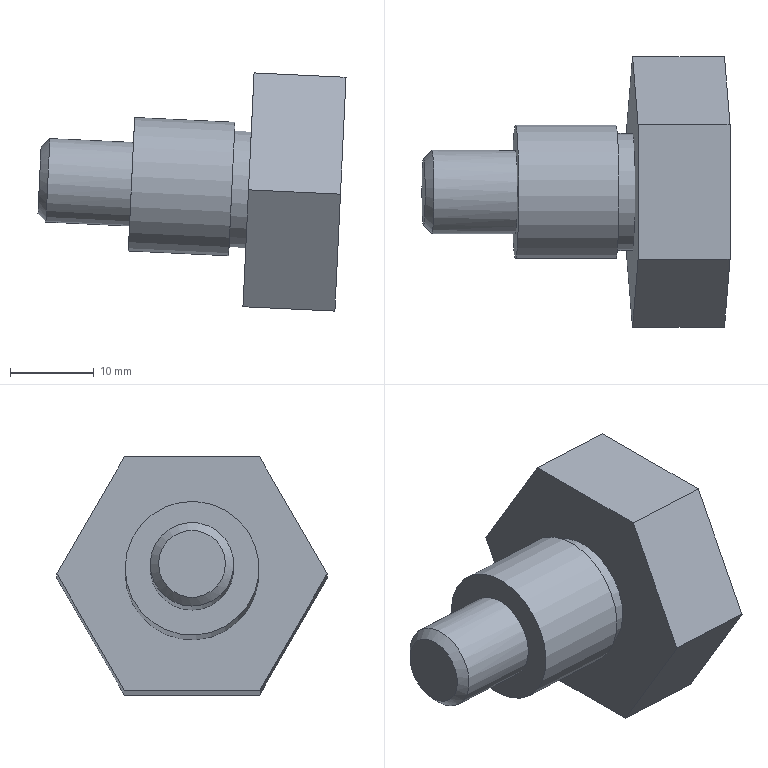Component | NX | SMALL_SHAFT | 1 solid | 15 faces | box 36.81 x 32.3 x 28.46 mm | volume 11024 mm3 | plane 11 | cylinder 3 | cone 1 | commonest cylinder face diameters 16 x1 10 x1 14 x1
STEP:
#1=CARTESIAN_POINT('',(0.,0.,0.));
#2=DIRECTION('',(0.,0.,1.));
#3=DIRECTION('',(1.,0.,0.));
#4=AXIS2_PLACEMENT_3D('',#1,#2,#3);
#5=CARTESIAN_POINT('',(20.177,-44.911,-1.909));
#6=VERTEX_POINT('',#5);
#7=CARTESIAN_POINT('',(20.507,-56.911,5.011));
#8=VERTEX_POINT('',#7);
#9=CARTESIAN_POINT('',(20.177,-52.911,-1.909));
#10=DIRECTION('',(-0.9989,0.,0.04757));
#11=DIRECTION('',(0.,1.,0.));
#12=AXIS2_PLACEMENT_3D('',#9,#10,#11);
#13=CIRCLE('',#12,8.);
#14=CARTESIAN_POINT('',(8.191,-52.911,-1.338));
#15=DIRECTION('',(0.9989,0.,-0.04757));
#16=DIRECTION('',(0.,-1.,0.));
#17=AXIS2_PLACEMENT_3D('',#14,#15,#16);
#18=CYLINDRICAL_SURFACE('',#17,8.);
#19=CARTESIAN_POINT('',(9.425,12.));
#20=DIRECTION('',(-1.,0.));
#21=VECTOR('',#20,1.);
#22=LINE('',#19,#21);
#23=(GEOMETRIC_REPRESENTATION_CONTEXT(2)PARAMETRIC_REPRESENTATION_CONTEXT()REPRESENTATION_CONTEXT('',''));
#24=DEFINITIONAL_REPRESENTATION('',(#22),#23);
#25=PCURVE('',#18,#24);
#26=CARTESIAN_POINT('',(20.51,-52.911,5.083));
#27=DIRECTION('',(-0.9989,0.,0.04757));
#28=DIRECTION('',(0.,1.,0.));
#29=AXIS2_PLACEMENT_3D('',#26,#27,#28);
#30=PLANE('',#29);
#31=CARTESIAN_POINT('',(0.,7.));
#32=DIRECTION('',(1.,0.));
#33=AXIS2_PLACEMENT_2D('',#31,#32);
#34=CIRCLE('',#33,8.);
#35=(GEOMETRIC_REPRESENTATION_CONTEXT(2)PARAMETRIC_REPRESENTATION_CONTEXT()REPRESENTATION_CONTEXT('',''));
#36=DEFINITIONAL_REPRESENTATION('',(#34),#35);
#37=PCURVE('',#30,#36);
#38=SURFACE_CURVE('',#13,(#25,#37),.PCURVE_S1.);
#39=EDGE_CURVE('',#6,#8,#38,.T.);
#40=ORIENTED_EDGE('',*,*,#39,.T.);
#41=CARTESIAN_POINT('',(8.521,-56.911,5.582));
#42=VERTEX_POINT('',#41);
#43=CARTESIAN_POINT('',(8.521,-56.911,5.582));
#44=CARTESIAN_POINT('',(20.507,-56.911,5.011));
#45=B_SPLINE_CURVE_WITH_KNOTS('',1,(#43,#44),.UNSPECIFIED.,.F.,.F.,(2,2),(0.,12.),.PIECEWISE_BEZIER_KNOTS.);
#46=CARTESIAN_POINT('',(5.236,0.));
#47=DIRECTION('',(0.,1.));
#48=VECTOR('',#47,1.);
#49=LINE('',#46,#48);
#50=(GEOMETRIC_REPRESENTATION_CONTEXT(2)PARAMETRIC_REPRESENTATION_CONTEXT()REPRESENTATION_CONTEXT('',''));
#51=DEFINITIONAL_REPRESENTATION('',(#49),#50);
#52=PCURVE('',#18,#51);
#53=CARTESIAN_POINT('',(11.519,0.));
#54=DIRECTION('',(0.,1.));
#55=VECTOR('',#54,1.);
#56=LINE('',#53,#55);
#57=(GEOMETRIC_REPRESENTATION_CONTEXT(2)PARAMETRIC_REPRESENTATION_CONTEXT()REPRESENTATION_CONTEXT('',''));
#58=DEFINITIONAL_REPRESENTATION('',(#56),#57);
#59=PCURVE('',#18,#58);
#60=SEAM_CURVE('',#45,(#52,#59),.PCURVE_S1.);
#61=EDGE_CURVE('',#42,#8,#60,.T.);
#62=ORIENTED_EDGE('',*,*,#61,.F.);
#63=CARTESIAN_POINT('',(8.191,-52.911,-1.338));
#64=DIRECTION('',(-0.9989,0.,0.04757));
#65=DIRECTION('',(0.0412,-0.5,0.865));
#66=AXIS2_PLACEMENT_3D('',#63,#64,#65);
#67=CIRCLE('',#66,8.);
#68=CARTESIAN_POINT('',(11.519,0.));
#69=DIRECTION('',(-1.,0.));
#70=VECTOR('',#69,1.);
#71=LINE('',#68,#70);
#72=(GEOMETRIC_REPRESENTATION_CONTEXT(2)PARAMETRIC_REPRESENTATION_CONTEXT()REPRESENTATION_CONTEXT('',''));
#73=DEFINITIONAL_REPRESENTATION('',(#71),#72);
#74=PCURVE('',#18,#73);
#75=CARTESIAN_POINT('',(8.191,-52.911,-1.338));
#76=DIRECTION('',(-0.9989,0.,0.04757));
#77=DIRECTION('',(0.,1.,0.));
#78=AXIS2_PLACEMENT_3D('',#75,#76,#77);
#79=PLANE('',#78);
#80=CARTESIAN_POINT('',(0.,0.));
#81=DIRECTION('',(-0.5,-0.866));
#82=AXIS2_PLACEMENT_2D('',#80,#81);
#83=CIRCLE('',#82,8.);
#84=(GEOMETRIC_REPRESENTATION_CONTEXT(2)PARAMETRIC_REPRESENTATION_CONTEXT()REPRESENTATION_CONTEXT('',''));
#85=DEFINITIONAL_REPRESENTATION('',(#83),#84);
#86=PCURVE('',#79,#85);
#87=SURFACE_CURVE('',#67,(#74,#86),.PCURVE_S1.);
#88=EDGE_CURVE('',#42,#42,#87,.T.);
#89=ORIENTED_EDGE('',*,*,#88,.F.);
#90=ORIENTED_EDGE('',*,*,#61,.T.);
#91=CARTESIAN_POINT('',(20.177,-52.911,-1.909));
#92=DIRECTION('',(-0.9989,0.,0.04757));
#93=DIRECTION('',(0.,1.,0.));
#94=AXIS2_PLACEMENT_3D('',#91,#92,#93);
#95=CIRCLE('',#94,8.);
#96=CARTESIAN_POINT('',(15.708,12.));
#97=DIRECTION('',(-1.,0.));
#98=VECTOR('',#97,1.);
#99=LINE('',#96,#98);
#100=(GEOMETRIC_REPRESENTATION_CONTEXT(2)PARAMETRIC_REPRESENTATION_CONTEXT()REPRESENTATION_CONTEXT('',''));
#101=DEFINITIONAL_REPRESENTATION('',(#99),#100);
#102=PCURVE('',#18,#101);
#103=CARTESIAN_POINT('',(0.,7.));
#104=DIRECTION('',(1.,0.));
#105=AXIS2_PLACEMENT_2D('',#103,#104);
#106=CIRCLE('',#105,8.);
#107=(GEOMETRIC_REPRESENTATION_CONTEXT(2)PARAMETRIC_REPRESENTATION_CONTEXT()REPRESENTATION_CONTEXT('',''));
#108=DEFINITIONAL_REPRESENTATION('',(#106),#107);
#109=PCURVE('',#30,#108);
#110=SURFACE_CURVE('',#95,(#102,#109),.PCURVE_S1.);
#111=EDGE_CURVE('',#8,#6,#110,.T.);
#112=ORIENTED_EDGE('',*,*,#111,.T.);
#113=EDGE_LOOP('',(#40,#62,#89,#90,#112));
#114=FACE_BOUND('',#113,.T.);
#115=ADVANCED_FACE('',(#114),#18,.T.);
#116=CARTESIAN_POINT('',(7.953,-52.911,-6.333));
#117=VERTEX_POINT('',#116);
#118=CARTESIAN_POINT('',(8.191,-52.911,-1.338));
#119=DIRECTION('',(-0.9989,0.,0.04757));
#120=DIRECTION('',(-0.04757,0.,-0.9989));
#121=AXIS2_PLACEMENT_3D('',#118,#119,#120);
#122=CIRCLE('',#121,5.);
#123=CARTESIAN_POINT('',(0.,0.));
#124=DIRECTION('',(0.,1.));
#125=AXIS2_PLACEMENT_2D('',#123,#124);
#126=CIRCLE('',#125,5.);
#127=(GEOMETRIC_REPRESENTATION_CONTEXT(2)PARAMETRIC_REPRESENTATION_CONTEXT()REPRESENTATION_CONTEXT('',''));
#128=DEFINITIONAL_REPRESENTATION('',(#126),#127);
#129=PCURVE('',#79,#128);
#130=CARTESIAN_POINT('',(-2.796,-52.911,-0.815));
#131=DIRECTION('',(0.9989,0.,-0.04757));
#132=DIRECTION('',(0.,-1.,0.));
#133=AXIS2_PLACEMENT_3D('',#130,#131,#132);
#134=CYLINDRICAL_SURFACE('',#133,5.);
#135=CARTESIAN_POINT('',(7.854,11.));
#136=DIRECTION('',(-1.,0.));
#137=VECTOR('',#136,1.);
#138=LINE('',#135,#137);
#139=(GEOMETRIC_REPRESENTATION_CONTEXT(2)PARAMETRIC_REPRESENTATION_CONTEXT()REPRESENTATION_CONTEXT('',''));
#140=DEFINITIONAL_REPRESENTATION('',(#138),#139);
#141=PCURVE('',#134,#140);
#142=SURFACE_CURVE('',#122,(#129,#141),.PCURVE_S1.);
#143=EDGE_CURVE('',#117,#117,#142,.T.);
#144=ORIENTED_EDGE('',*,*,#143,.F.);
#145=EDGE_LOOP('',(#144));
#146=FACE_BOUND('',#145,.T.);
#147=ORIENTED_EDGE('',*,*,#88,.T.);
#148=EDGE_LOOP('',(#147));
#149=FACE_BOUND('',#148,.T.);
#150=ADVANCED_FACE('',(#146,#149),#79,.T.);
#151=CARTESIAN_POINT('',(-1.798,-47.911,-0.8626));
#152=VERTEX_POINT('',#151);
#153=CARTESIAN_POINT('',(-2.035,-52.911,-5.857));
#154=VERTEX_POINT('',#153);
#155=CARTESIAN_POINT('',(-1.798,-52.911,-0.8626));
#156=DIRECTION('',(0.9989,0.,-0.04757));
#157=DIRECTION('',(0.,1.,0.));
#158=AXIS2_PLACEMENT_3D('',#155,#156,#157);
#159=CIRCLE('',#158,5.);
#160=CARTESIAN_POINT('',(3.142,1.));
#161=DIRECTION('',(1.,0.));
#162=VECTOR('',#161,1.);
#163=LINE('',#160,#162);
#164=(GEOMETRIC_REPRESENTATION_CONTEXT(2)PARAMETRIC_REPRESENTATION_CONTEXT()REPRESENTATION_CONTEXT('',''));
#165=DEFINITIONAL_REPRESENTATION('',(#163),#164);
#166=PCURVE('',#134,#165);
#167=CARTESIAN_POINT('',(-2.796,-52.911,-0.815));
#168=DIRECTION('',(0.9989,0.,-0.04757));
#169=DIRECTION('',(0.,-1.,0.));
#170=AXIS2_PLACEMENT_3D('',#167,#168,#169);
#171=CONICAL_SURFACE('',#170,4.,0.7854);
#172=CARTESIAN_POINT('',(3.142,1.));
#173=DIRECTION('',(1.,0.));
#174=VECTOR('',#173,1.);
#175=LINE('',#172,#174);
#176=(GEOMETRIC_REPRESENTATION_CONTEXT(2)PARAMETRIC_REPRESENTATION_CONTEXT()REPRESENTATION_CONTEXT('',''));
#177=DEFINITIONAL_REPRESENTATION('',(#175),#176);
#178=PCURVE('',#171,#177);
#179=SURFACE_CURVE('',#159,(#166,#178),.PCURVE_S1.);
#180=EDGE_CURVE('',#152,#154,#179,.T.);
#181=ORIENTED_EDGE('',*,*,#180,.T.);
#182=CARTESIAN_POINT('',(-2.035,-52.911,-5.857));
#183=CARTESIAN_POINT('',(7.953,-52.911,-6.333));
#184=B_SPLINE_CURVE_WITH_KNOTS('',1,(#182,#183),.UNSPECIFIED.,.F.,.F.,(2,2),(1.,11.),.PIECEWISE_BEZIER_KNOTS.);
#185=CARTESIAN_POINT('',(7.854,0.));
#186=DIRECTION('',(0.,1.));
#187=VECTOR('',#186,1.);
#188=LINE('',#185,#187);
#189=(GEOMETRIC_REPRESENTATION_CONTEXT(2)PARAMETRIC_REPRESENTATION_CONTEXT()REPRESENTATION_CONTEXT('',''));
#190=DEFINITIONAL_REPRESENTATION('',(#188),#189);
#191=PCURVE('',#134,#190);
#192=CARTESIAN_POINT('',(1.571,0.));
#193=DIRECTION('',(0.,1.));
#194=VECTOR('',#193,1.);
#195=LINE('',#192,#194);
#196=(GEOMETRIC_REPRESENTATION_CONTEXT(2)PARAMETRIC_REPRESENTATION_CONTEXT()REPRESENTATION_CONTEXT('',''));
#197=DEFINITIONAL_REPRESENTATION('',(#195),#196);
#198=PCURVE('',#134,#197);
#199=SEAM_CURVE('',#184,(#191,#198),.PCURVE_S1.);
#200=EDGE_CURVE('',#154,#117,#199,.T.);
#201=ORIENTED_EDGE('',*,*,#200,.T.);
#202=ORIENTED_EDGE('',*,*,#143,.T.);
#203=ORIENTED_EDGE('',*,*,#200,.F.);
#204=CARTESIAN_POINT('',(-1.798,-52.911,-0.8626));
#205=DIRECTION('',(0.9989,0.,-0.04757));
#206=DIRECTION('',(0.,1.,0.));
#207=AXIS2_PLACEMENT_3D('',#204,#205,#206);
#208=CIRCLE('',#207,5.);
#209=CARTESIAN_POINT('',(-3.142,1.));
#210=DIRECTION('',(1.,0.));
#211=VECTOR('',#210,1.);
#212=LINE('',#209,#211);
#213=(GEOMETRIC_REPRESENTATION_CONTEXT(2)PARAMETRIC_REPRESENTATION_CONTEXT()REPRESENTATION_CONTEXT('',''));
#214=DEFINITIONAL_REPRESENTATION('',(#212),#213);
#215=PCURVE('',#134,#214);
#216=CARTESIAN_POINT('',(3.142,1.));
#217=DIRECTION('',(1.,-0.));
#218=VECTOR('',#217,1.);
#219=LINE('',#216,#218);
#220=(GEOMETRIC_REPRESENTATION_CONTEXT(2)PARAMETRIC_REPRESENTATION_CONTEXT()REPRESENTATION_CONTEXT('',''));
#221=DEFINITIONAL_REPRESENTATION('',(#219),#220);
#222=PCURVE('',#171,#221);
#223=SURFACE_CURVE('',#208,(#215,#222),.PCURVE_S1.);
#224=EDGE_CURVE('',#154,#152,#223,.T.);
#225=ORIENTED_EDGE('',*,*,#224,.T.);
#226=EDGE_LOOP('',(#181,#201,#202,#203,#225));
#227=FACE_BOUND('',#226,.T.);
#228=ADVANCED_FACE('',(#227),#134,.T.);
#229=CARTESIAN_POINT('',(-2.796,-48.911,-0.815));
#230=VERTEX_POINT('',#229);
#231=CARTESIAN_POINT('',(-2.796,-52.911,-0.815));
#232=DIRECTION('',(-0.9989,0.,0.04757));
#233=DIRECTION('',(0.,1.,0.));
#234=AXIS2_PLACEMENT_3D('',#231,#232,#233);
#235=CIRCLE('',#234,4.);
#236=CARTESIAN_POINT('',(-2.796,-52.911,-0.815));
#237=DIRECTION('',(-0.9989,0.,0.04757));
#238=DIRECTION('',(0.,1.,0.));
#239=AXIS2_PLACEMENT_3D('',#236,#237,#238);
#240=PLANE('',#239);
#241=CARTESIAN_POINT('',(0.,0.));
#242=DIRECTION('',(1.,0.));
#243=AXIS2_PLACEMENT_2D('',#241,#242);
#244=CIRCLE('',#243,4.);
#245=(GEOMETRIC_REPRESENTATION_CONTEXT(2)PARAMETRIC_REPRESENTATION_CONTEXT()REPRESENTATION_CONTEXT('',''));
#246=DEFINITIONAL_REPRESENTATION('',(#244),#245);
#247=PCURVE('',#240,#246);
#248=CARTESIAN_POINT('',(9.425,0.));
#249=DIRECTION('',(-1.,0.));
#250=VECTOR('',#249,1.);
#251=LINE('',#248,#250);
#252=(GEOMETRIC_REPRESENTATION_CONTEXT(2)PARAMETRIC_REPRESENTATION_CONTEXT()REPRESENTATION_CONTEXT('',''));
#253=DEFINITIONAL_REPRESENTATION('',(#251),#252);
#254=PCURVE('',#171,#253);
#255=SURFACE_CURVE('',#235,(#247,#254),.PCURVE_S1.);
#256=EDGE_CURVE('',#230,#230,#255,.T.);
#257=ORIENTED_EDGE('',*,*,#256,.T.);
#258=EDGE_LOOP('',(#257));
#259=FACE_BOUND('',#258,.T.);
#260=ADVANCED_FACE('',(#259),#240,.T.);
#261=ORIENTED_EDGE('',*,*,#180,.F.);
#262=CARTESIAN_POINT('',(-2.796,-48.911,-0.815));
#263=CARTESIAN_POINT('',(-1.798,-47.911,-0.8626));
#264=B_SPLINE_CURVE_WITH_KNOTS('',1,(#262,#263),.UNSPECIFIED.,.F.,.F.,(2,2),(0.,1.414),.PIECEWISE_BEZIER_KNOTS.);
#265=CARTESIAN_POINT('',(3.142,0.));
#266=DIRECTION('',(0.,1.));
#267=VECTOR('',#266,1.);
#268=LINE('',#265,#267);
#269=(GEOMETRIC_REPRESENTATION_CONTEXT(2)PARAMETRIC_REPRESENTATION_CONTEXT()REPRESENTATION_CONTEXT('',''));
#270=DEFINITIONAL_REPRESENTATION('',(#268),#269);
#271=PCURVE('',#171,#270);
#272=CARTESIAN_POINT('',(9.425,0.));
#273=DIRECTION('',(0.,1.));
#274=VECTOR('',#273,1.);
#275=LINE('',#272,#274);
#276=(GEOMETRIC_REPRESENTATION_CONTEXT(2)PARAMETRIC_REPRESENTATION_CONTEXT()REPRESENTATION_CONTEXT('',''));
#277=DEFINITIONAL_REPRESENTATION('',(#275),#276);
#278=PCURVE('',#171,#277);
#279=SEAM_CURVE('',#264,(#271,#278),.PCURVE_S1.);
#280=EDGE_CURVE('',#230,#152,#279,.T.);
#281=ORIENTED_EDGE('',*,*,#280,.F.);
#282=ORIENTED_EDGE('',*,*,#256,.F.);
#283=ORIENTED_EDGE('',*,*,#280,.T.);
#284=ORIENTED_EDGE('',*,*,#224,.F.);
#285=EDGE_LOOP('',(#261,#281,#282,#283,#284));
#286=FACE_BOUND('',#285,.T.);
#287=ADVANCED_FACE('',(#286),#171,.T.);
#288=CARTESIAN_POINT('',(20.177,-45.911,-1.909));
#289=VERTEX_POINT('',#288);
#290=CARTESIAN_POINT('',(20.177,-52.911,-1.909));
#291=DIRECTION('',(0.9989,0.,-0.04757));
#292=DIRECTION('',(0.,1.,0.));
#293=AXIS2_PLACEMENT_3D('',#290,#291,#292);
#294=CIRCLE('',#293,7.);
#295=CARTESIAN_POINT('',(8.191,-52.911,-1.338));
#296=DIRECTION('',(-0.9989,0.,0.04757));
#297=DIRECTION('',(0.,1.,0.));
#298=AXIS2_PLACEMENT_3D('',#295,#296,#297);
#299=CYLINDRICAL_SURFACE('',#298,7.);
#300=CARTESIAN_POINT('',(6.283,-12.));
#301=DIRECTION('',(-1.,0.));
#302=VECTOR('',#301,1.);
#303=LINE('',#300,#302);
#304=(GEOMETRIC_REPRESENTATION_CONTEXT(2)PARAMETRIC_REPRESENTATION_CONTEXT()REPRESENTATION_CONTEXT('',''));
#305=DEFINITIONAL_REPRESENTATION('',(#303),#304);
#306=PCURVE('',#299,#305);
#307=CARTESIAN_POINT('',(7.,7.));
#308=CARTESIAN_POINT('',(7.,-5.124));
#309=CARTESIAN_POINT('',(-3.5,0.9378));
#310=CARTESIAN_POINT('',(-14.,7.));
#311=CARTESIAN_POINT('',(-3.5,13.062));
#312=CARTESIAN_POINT('',(7.,19.124));
#313=CARTESIAN_POINT('',(7.,7.));
#314=(BOUNDED_CURVE()B_SPLINE_CURVE(2,(#307,#308,#309,#310,#311,#312,#313),.UNSPECIFIED.,.T.,.F.)B_SPLINE_CURVE_WITH_KNOTS((1,2,2,2,2,1),(-2.094,0.,2.094,4.189,6.283,8.378),.UNSPECIFIED.)CURVE()GEOMETRIC_REPRESENTATION_ITEM()RATIONAL_B_SPLINE_CURVE((1.,0.5,1.,0.5,1.,0.5,1.))REPRESENTATION_ITEM(''));
#315=(GEOMETRIC_REPRESENTATION_CONTEXT(2)PARAMETRIC_REPRESENTATION_CONTEXT()REPRESENTATION_CONTEXT('',''));
#316=DEFINITIONAL_REPRESENTATION('',(#314),#315);
#317=PCURVE('',#30,#316);
#318=SURFACE_CURVE('',#294,(#306,#317),.PCURVE_S1.);
#319=EDGE_CURVE('',#289,#289,#318,.T.);
#320=ORIENTED_EDGE('',*,*,#319,.T.);
#321=CARTESIAN_POINT('',(22.175,-45.911,-2.004));
#322=VERTEX_POINT('',#321);
#323=CARTESIAN_POINT('',(22.175,-45.911,-2.004));
#324=CARTESIAN_POINT('',(20.177,-45.911,-1.909));
#325=B_SPLINE_CURVE_WITH_KNOTS('',1,(#323,#324),.UNSPECIFIED.,.F.,.F.,(2,2),(-14.,-12.),.PIECEWISE_BEZIER_KNOTS.);
#326=CARTESIAN_POINT('',(0.,0.));
#327=DIRECTION('',(0.,1.));
#328=VECTOR('',#327,1.);
#329=LINE('',#326,#328);
#330=(GEOMETRIC_REPRESENTATION_CONTEXT(2)PARAMETRIC_REPRESENTATION_CONTEXT()REPRESENTATION_CONTEXT('',''));
#331=DEFINITIONAL_REPRESENTATION('',(#329),#330);
#332=PCURVE('',#299,#331);
#333=CARTESIAN_POINT('',(6.283,0.));
#334=DIRECTION('',(0.,1.));
#335=VECTOR('',#334,1.);
#336=LINE('',#333,#335);
#337=(GEOMETRIC_REPRESENTATION_CONTEXT(2)PARAMETRIC_REPRESENTATION_CONTEXT()REPRESENTATION_CONTEXT('',''));
#338=DEFINITIONAL_REPRESENTATION('',(#336),#337);
#339=PCURVE('',#299,#338);
#340=SEAM_CURVE('',#325,(#332,#339),.PCURVE_S1.);
#341=EDGE_CURVE('',#322,#289,#340,.T.);
#342=ORIENTED_EDGE('',*,*,#341,.F.);
#343=CARTESIAN_POINT('',(22.175,-52.911,-2.004));
#344=DIRECTION('',(-0.9989,0.,0.04757));
#345=DIRECTION('',(0.,1.,0.));
#346=AXIS2_PLACEMENT_3D('',#343,#344,#345);
#347=CIRCLE('',#346,7.);
#348=CARTESIAN_POINT('',(0.,-14.));
#349=DIRECTION('',(1.,0.));
#350=VECTOR('',#349,1.);
#351=LINE('',#348,#350);
#352=(GEOMETRIC_REPRESENTATION_CONTEXT(2)PARAMETRIC_REPRESENTATION_CONTEXT()REPRESENTATION_CONTEXT('',''));
#353=DEFINITIONAL_REPRESENTATION('',(#351),#352);
#354=PCURVE('',#299,#353);
#355=CARTESIAN_POINT('',(22.175,-52.911,-2.004));
#356=DIRECTION('',(0.9989,0.,-0.04757));
#357=DIRECTION('',(0.,-1.,0.));
#358=AXIS2_PLACEMENT_3D('',#355,#356,#357);
#359=PLANE('',#358);
#360=CARTESIAN_POINT('',(-7.,0.));
#361=CARTESIAN_POINT('',(-7.,12.124));
#362=CARTESIAN_POINT('',(3.5,6.062));
#363=CARTESIAN_POINT('',(14.,0.));
#364=CARTESIAN_POINT('',(3.5,-6.062));
#365=CARTESIAN_POINT('',(-7.,-12.124));
#366=CARTESIAN_POINT('',(-7.,0.));
#367=(BOUNDED_CURVE()B_SPLINE_CURVE(2,(#360,#361,#362,#363,#364,#365,#366),.UNSPECIFIED.,.T.,.F.)B_SPLINE_CURVE_WITH_KNOTS((1,2,2,2,2,1),(-2.094,0.,2.094,4.189,6.283,8.378),.UNSPECIFIED.)CURVE()GEOMETRIC_REPRESENTATION_ITEM()RATIONAL_B_SPLINE_CURVE((1.,0.5,1.,0.5,1.,0.5,1.))REPRESENTATION_ITEM(''));
#368=(GEOMETRIC_REPRESENTATION_CONTEXT(2)PARAMETRIC_REPRESENTATION_CONTEXT()REPRESENTATION_CONTEXT('',''));
#369=DEFINITIONAL_REPRESENTATION('',(#367),#368);
#370=PCURVE('',#359,#369);
#371=SURFACE_CURVE('',#347,(#354,#370),.PCURVE_S1.);
#372=EDGE_CURVE('',#322,#322,#371,.T.);
#373=ORIENTED_EDGE('',*,*,#372,.T.);
#374=ORIENTED_EDGE('',*,*,#341,.T.);
#375=EDGE_LOOP('',(#320,#342,#373,#374));
#376=FACE_BOUND('',#375,.T.);
#377=ADVANCED_FACE('',(#376),#299,.T.);
#378=ORIENTED_EDGE('',*,*,#39,.F.);
#379=ORIENTED_EDGE('',*,*,#111,.F.);
#380=EDGE_LOOP('',(#378,#379));
#381=FACE_BOUND('',#380,.T.);
#382=ORIENTED_EDGE('',*,*,#319,.F.);
#383=EDGE_LOOP('',(#382));
#384=FACE_BOUND('',#383,.T.);
#385=ADVANCED_FACE('',(#381,#384),#30,.F.);
#386=CARTESIAN_POINT('',(33.828,-44.836,11.443));
#387=VERTEX_POINT('',#386);
#388=CARTESIAN_POINT('',(33.828,-60.986,11.443));
#389=VERTEX_POINT('',#388);
#390=CARTESIAN_POINT('',(33.828,-44.836,11.443));
#391=DIRECTION('',(0.,-1.,0.));
#392=VECTOR('',#391,1.);
#393=LINE('',#390,#392);
#394=CARTESIAN_POINT('',(33.163,-52.911,-2.528));
#395=DIRECTION('',(0.9989,0.,-0.04757));
#396=DIRECTION('',(0.,-1.,0.));
#397=AXIS2_PLACEMENT_3D('',#394,#395,#396);
#398=PLANE('',#397);
#399=CARTESIAN_POINT('',(-8.075,-13.986));
#400=DIRECTION('',(1.,-0.));
#401=VECTOR('',#400,1.);
#402=LINE('',#399,#401);
#403=(GEOMETRIC_REPRESENTATION_CONTEXT(2)PARAMETRIC_REPRESENTATION_CONTEXT()REPRESENTATION_CONTEXT('',''));
#404=DEFINITIONAL_REPRESENTATION('',(#402),#403);
#405=PCURVE('',#398,#404);
#406=CARTESIAN_POINT('',(33.828,-44.836,11.443));
#407=DIRECTION('',(-0.04757,-0.,-0.9989));
#408=DIRECTION('',(0.,-1.,0.));
#409=AXIS2_PLACEMENT_3D('',#406,#407,#408);
#410=PLANE('',#409);
#411=CARTESIAN_POINT('',(0.,0.));
#412=DIRECTION('',(1.,0.));
#413=VECTOR('',#412,1.);
#414=LINE('',#411,#413);
#415=(GEOMETRIC_REPRESENTATION_CONTEXT(2)PARAMETRIC_REPRESENTATION_CONTEXT()REPRESENTATION_CONTEXT('',''));
#416=DEFINITIONAL_REPRESENTATION('',(#414),#415);
#417=PCURVE('',#410,#416);
#418=SURFACE_CURVE('',#393,(#405,#417),.PCURVE_S1.);
#419=EDGE_CURVE('',#387,#389,#418,.T.);
#420=ORIENTED_EDGE('',*,*,#419,.T.);
#421=CARTESIAN_POINT('',(33.163,-69.061,-2.528));
#422=VERTEX_POINT('',#421);
#423=CARTESIAN_POINT('',(33.828,-60.986,11.443));
#424=DIRECTION('',(-0.0412,-0.5,-0.865));
#425=VECTOR('',#424,1.);
#426=LINE('',#423,#425);
#427=CARTESIAN_POINT('',(8.075,-13.986));
#428=DIRECTION('',(0.5,0.866));
#429=VECTOR('',#428,1.);
#430=LINE('',#427,#429);
#431=(GEOMETRIC_REPRESENTATION_CONTEXT(2)PARAMETRIC_REPRESENTATION_CONTEXT()REPRESENTATION_CONTEXT('',''));
#432=DEFINITIONAL_REPRESENTATION('',(#430),#431);
#433=PCURVE('',#398,#432);
#434=CARTESIAN_POINT('',(33.828,-60.986,11.443));
#435=DIRECTION('',(-0.02378,0.866,-0.4994));
#436=DIRECTION('',(-0.0412,-0.5,-0.865));
#437=AXIS2_PLACEMENT_3D('',#434,#435,#436);
#438=PLANE('',#437);
#439=CARTESIAN_POINT('',(0.,0.));
#440=DIRECTION('',(1.,0.));
#441=VECTOR('',#440,1.);
#442=LINE('',#439,#441);
#443=(GEOMETRIC_REPRESENTATION_CONTEXT(2)PARAMETRIC_REPRESENTATION_CONTEXT()REPRESENTATION_CONTEXT('',''));
#444=DEFINITIONAL_REPRESENTATION('',(#442),#443);
#445=PCURVE('',#438,#444);
#446=SURFACE_CURVE('',#426,(#433,#445),.PCURVE_S1.);
#447=EDGE_CURVE('',#389,#422,#446,.T.);
#448=ORIENTED_EDGE('',*,*,#447,.T.);
#449=CARTESIAN_POINT('',(32.497,-60.986,-16.498));
#450=VERTEX_POINT('',#449);
#451=CARTESIAN_POINT('',(33.163,-69.061,-2.528));
#452=DIRECTION('',(-0.0412,0.5,-0.865));
#453=VECTOR('',#452,1.);
#454=LINE('',#451,#453);
#455=CARTESIAN_POINT('',(16.15,-0.));
#456=DIRECTION('',(-0.5,0.866));
#457=VECTOR('',#456,1.);
#458=LINE('',#455,#457);
#459=(GEOMETRIC_REPRESENTATION_CONTEXT(2)PARAMETRIC_REPRESENTATION_CONTEXT()REPRESENTATION_CONTEXT('',''));
#460=DEFINITIONAL_REPRESENTATION('',(#458),#459);
#461=PCURVE('',#398,#460);
#462=CARTESIAN_POINT('',(33.163,-69.061,-2.528));
#463=DIRECTION('',(0.02378,0.866,0.4994));
#464=DIRECTION('',(-0.0412,0.5,-0.865));
#465=AXIS2_PLACEMENT_3D('',#462,#463,#464);
#466=PLANE('',#465);
#467=CARTESIAN_POINT('',(0.,0.));
#468=DIRECTION('',(1.,0.));
#469=VECTOR('',#468,1.);
#470=LINE('',#467,#469);
#471=(GEOMETRIC_REPRESENTATION_CONTEXT(2)PARAMETRIC_REPRESENTATION_CONTEXT()REPRESENTATION_CONTEXT('',''));
#472=DEFINITIONAL_REPRESENTATION('',(#470),#471);
#473=PCURVE('',#466,#472);
#474=SURFACE_CURVE('',#454,(#461,#473),.PCURVE_S1.);
#475=EDGE_CURVE('',#422,#450,#474,.T.);
#476=ORIENTED_EDGE('',*,*,#475,.T.);
#477=CARTESIAN_POINT('',(32.497,-44.836,-16.498));
#478=VERTEX_POINT('',#477);
#479=CARTESIAN_POINT('',(32.497,-60.986,-16.498));
#480=DIRECTION('',(0.,1.,0.));
#481=VECTOR('',#480,1.);
#482=LINE('',#479,#481);
#483=CARTESIAN_POINT('',(8.075,13.986));
#484=DIRECTION('',(-1.,-0.));
#485=VECTOR('',#484,1.);
#486=LINE('',#483,#485);
#487=(GEOMETRIC_REPRESENTATION_CONTEXT(2)PARAMETRIC_REPRESENTATION_CONTEXT()REPRESENTATION_CONTEXT('',''));
#488=DEFINITIONAL_REPRESENTATION('',(#486),#487);
#489=PCURVE('',#398,#488);
#490=CARTESIAN_POINT('',(32.497,-60.986,-16.498));
#491=DIRECTION('',(0.04757,-0.,0.9989));
#492=DIRECTION('',(0.,1.,0.));
#493=AXIS2_PLACEMENT_3D('',#490,#491,#492);
#494=PLANE('',#493);
#495=CARTESIAN_POINT('',(0.,0.));
#496=DIRECTION('',(1.,0.));
#497=VECTOR('',#496,1.);
#498=LINE('',#495,#497);
#499=(GEOMETRIC_REPRESENTATION_CONTEXT(2)PARAMETRIC_REPRESENTATION_CONTEXT()REPRESENTATION_CONTEXT('',''));
#500=DEFINITIONAL_REPRESENTATION('',(#498),#499);
#501=PCURVE('',#494,#500);
#502=SURFACE_CURVE('',#482,(#489,#501),.PCURVE_S1.);
#503=EDGE_CURVE('',#450,#478,#502,.T.);
#504=ORIENTED_EDGE('',*,*,#503,.T.);
#505=CARTESIAN_POINT('',(33.163,-36.761,-2.528));
#506=VERTEX_POINT('',#505);
#507=CARTESIAN_POINT('',(32.497,-44.836,-16.498));
#508=DIRECTION('',(0.0412,0.5,0.865));
#509=VECTOR('',#508,1.);
#510=LINE('',#507,#509);
#511=CARTESIAN_POINT('',(-8.075,13.986));
#512=DIRECTION('',(-0.5,-0.866));
#513=VECTOR('',#512,1.);
#514=LINE('',#511,#513);
#515=(GEOMETRIC_REPRESENTATION_CONTEXT(2)PARAMETRIC_REPRESENTATION_CONTEXT()REPRESENTATION_CONTEXT('',''));
#516=DEFINITIONAL_REPRESENTATION('',(#514),#515);
#517=PCURVE('',#398,#516);
#518=CARTESIAN_POINT('',(32.497,-44.836,-16.498));
#519=DIRECTION('',(0.02378,-0.866,0.4994));
#520=DIRECTION('',(0.0412,0.5,0.865));
#521=AXIS2_PLACEMENT_3D('',#518,#519,#520);
#522=PLANE('',#521);
#523=CARTESIAN_POINT('',(0.,0.));
#524=DIRECTION('',(1.,0.));
#525=VECTOR('',#524,1.);
#526=LINE('',#523,#525);
#527=(GEOMETRIC_REPRESENTATION_CONTEXT(2)PARAMETRIC_REPRESENTATION_CONTEXT()REPRESENTATION_CONTEXT('',''));
#528=DEFINITIONAL_REPRESENTATION('',(#526),#527);
#529=PCURVE('',#522,#528);
#530=SURFACE_CURVE('',#510,(#517,#529),.PCURVE_S1.);
#531=EDGE_CURVE('',#478,#506,#530,.T.);
#532=ORIENTED_EDGE('',*,*,#531,.T.);
#533=CARTESIAN_POINT('',(33.163,-36.761,-2.528));
#534=DIRECTION('',(0.0412,-0.5,0.865));
#535=VECTOR('',#534,1.);
#536=LINE('',#533,#535);
#537=CARTESIAN_POINT('',(-16.15,0.));
#538=DIRECTION('',(0.5,-0.866));
#539=VECTOR('',#538,1.);
#540=LINE('',#537,#539);
#541=(GEOMETRIC_REPRESENTATION_CONTEXT(2)PARAMETRIC_REPRESENTATION_CONTEXT()REPRESENTATION_CONTEXT('',''));
#542=DEFINITIONAL_REPRESENTATION('',(#540),#541);
#543=PCURVE('',#398,#542);
#544=CARTESIAN_POINT('',(33.163,-36.761,-2.528));
#545=DIRECTION('',(-0.02378,-0.866,-0.4994));
#546=DIRECTION('',(0.0412,-0.5,0.865));
#547=AXIS2_PLACEMENT_3D('',#544,#545,#546);
#548=PLANE('',#547);
#549=CARTESIAN_POINT('',(0.,0.));
#550=DIRECTION('',(1.,-0.));
#551=VECTOR('',#550,1.);
#552=LINE('',#549,#551);
#553=(GEOMETRIC_REPRESENTATION_CONTEXT(2)PARAMETRIC_REPRESENTATION_CONTEXT()REPRESENTATION_CONTEXT('',''));
#554=DEFINITIONAL_REPRESENTATION('',(#552),#553);
#555=PCURVE('',#548,#554);
#556=SURFACE_CURVE('',#536,(#543,#555),.PCURVE_S1.);
#557=EDGE_CURVE('',#506,#387,#556,.T.);
#558=ORIENTED_EDGE('',*,*,#557,.T.);
#559=EDGE_LOOP('',(#420,#448,#476,#504,#532,#558));
#560=FACE_BOUND('',#559,.T.);
#561=ADVANCED_FACE('',(#560),#398,.T.);
#562=CARTESIAN_POINT('',(22.841,-60.986,11.966));
#563=VERTEX_POINT('',#562);
#564=CARTESIAN_POINT('',(22.175,-69.061,-2.004));
#565=VERTEX_POINT('',#564);
#566=CARTESIAN_POINT('',(22.841,-60.986,11.966));
#567=DIRECTION('',(-0.0412,-0.5,-0.865));
#568=VECTOR('',#567,1.);
#569=LINE('',#566,#568);
#570=CARTESIAN_POINT('',(-0.,11.));
#571=DIRECTION('',(1.,0.));
#572=VECTOR('',#571,1.);
#573=LINE('',#570,#572);
#574=(GEOMETRIC_REPRESENTATION_CONTEXT(2)PARAMETRIC_REPRESENTATION_CONTEXT()REPRESENTATION_CONTEXT('',''));
#575=DEFINITIONAL_REPRESENTATION('',(#573),#574);
#576=PCURVE('',#438,#575);
#577=CARTESIAN_POINT('',(8.075,-13.986));
#578=DIRECTION('',(0.5,0.866));
#579=VECTOR('',#578,1.);
#580=LINE('',#577,#579);
#581=(GEOMETRIC_REPRESENTATION_CONTEXT(2)PARAMETRIC_REPRESENTATION_CONTEXT()REPRESENTATION_CONTEXT('',''));
#582=DEFINITIONAL_REPRESENTATION('',(#580),#581);
#583=PCURVE('',#359,#582);
#584=SURFACE_CURVE('',#569,(#576,#583),.PCURVE_S1.);
#585=EDGE_CURVE('',#563,#565,#584,.T.);
#586=ORIENTED_EDGE('',*,*,#585,.T.);
#587=CARTESIAN_POINT('',(33.163,-69.061,-2.528));
#588=DIRECTION('',(-0.9989,0.,0.04757));
#589=VECTOR('',#588,1.);
#590=LINE('',#587,#589);
#591=CARTESIAN_POINT('',(16.15,0.));
#592=DIRECTION('',(0.,1.));
#593=VECTOR('',#592,1.);
#594=LINE('',#591,#593);
#595=(GEOMETRIC_REPRESENTATION_CONTEXT(2)PARAMETRIC_REPRESENTATION_CONTEXT()REPRESENTATION_CONTEXT('',''));
#596=DEFINITIONAL_REPRESENTATION('',(#594),#595);
#597=PCURVE('',#438,#596);
#598=CARTESIAN_POINT('',(0.,-0.));
#599=DIRECTION('',(0.,1.));
#600=VECTOR('',#599,1.);
#601=LINE('',#598,#600);
#602=(GEOMETRIC_REPRESENTATION_CONTEXT(2)PARAMETRIC_REPRESENTATION_CONTEXT()REPRESENTATION_CONTEXT('',''));
#603=DEFINITIONAL_REPRESENTATION('',(#601),#602);
#604=PCURVE('',#466,#603);
#605=SURFACE_CURVE('',#590,(#597,#604),.PCURVE_S1.);
#606=EDGE_CURVE('',#422,#565,#605,.T.);
#607=ORIENTED_EDGE('',*,*,#606,.F.);
#608=ORIENTED_EDGE('',*,*,#447,.F.);
#609=CARTESIAN_POINT('',(33.828,-60.986,11.443));
#610=DIRECTION('',(-0.9989,0.,0.04757));
#611=VECTOR('',#610,1.);
#612=LINE('',#609,#611);
#613=CARTESIAN_POINT('',(0.,0.));
#614=DIRECTION('',(0.,1.));
#615=VECTOR('',#614,1.);
#616=LINE('',#613,#615);
#617=(GEOMETRIC_REPRESENTATION_CONTEXT(2)PARAMETRIC_REPRESENTATION_CONTEXT()REPRESENTATION_CONTEXT('',''));
#618=DEFINITIONAL_REPRESENTATION('',(#616),#617);
#619=PCURVE('',#438,#618);
#620=CARTESIAN_POINT('',(16.15,0.));
#621=DIRECTION('',(-0.,1.));
#622=VECTOR('',#621,1.);
#623=LINE('',#620,#622);
#624=(GEOMETRIC_REPRESENTATION_CONTEXT(2)PARAMETRIC_REPRESENTATION_CONTEXT()REPRESENTATION_CONTEXT('',''));
#625=DEFINITIONAL_REPRESENTATION('',(#623),#624);
#626=PCURVE('',#410,#625);
#627=SURFACE_CURVE('',#612,(#619,#626),.PCURVE_S1.);
#628=EDGE_CURVE('',#389,#563,#627,.T.);
#629=ORIENTED_EDGE('',*,*,#628,.T.);
#630=EDGE_LOOP('',(#586,#607,#608,#629));
#631=FACE_BOUND('',#630,.T.);
#632=ADVANCED_FACE('',(#631),#438,.F.);
#633=CARTESIAN_POINT('',(21.51,-60.986,-15.975));
#634=VERTEX_POINT('',#633);
#635=CARTESIAN_POINT('',(22.175,-69.061,-2.004));
#636=DIRECTION('',(-0.0412,0.5,-0.865));
#637=VECTOR('',#636,1.);
#638=LINE('',#635,#637);
#639=CARTESIAN_POINT('',(0.,11.));
#640=DIRECTION('',(1.,0.));
#641=VECTOR('',#640,1.);
#642=LINE('',#639,#641);
#643=(GEOMETRIC_REPRESENTATION_CONTEXT(2)PARAMETRIC_REPRESENTATION_CONTEXT()REPRESENTATION_CONTEXT('',''));
#644=DEFINITIONAL_REPRESENTATION('',(#642),#643);
#645=PCURVE('',#466,#644);
#646=CARTESIAN_POINT('',(16.15,-0.));
#647=DIRECTION('',(-0.5,0.866));
#648=VECTOR('',#647,1.);
#649=LINE('',#646,#648);
#650=(GEOMETRIC_REPRESENTATION_CONTEXT(2)PARAMETRIC_REPRESENTATION_CONTEXT()REPRESENTATION_CONTEXT('',''));
#651=DEFINITIONAL_REPRESENTATION('',(#649),#650);
#652=PCURVE('',#359,#651);
#653=SURFACE_CURVE('',#638,(#645,#652),.PCURVE_S1.);
#654=EDGE_CURVE('',#565,#634,#653,.T.);
#655=ORIENTED_EDGE('',*,*,#654,.T.);
#656=CARTESIAN_POINT('',(32.497,-60.986,-16.498));
#657=DIRECTION('',(-0.9989,0.,0.04757));
#658=VECTOR('',#657,1.);
#659=LINE('',#656,#658);
#660=CARTESIAN_POINT('',(16.15,-0.));
#661=DIRECTION('',(0.,1.));
#662=VECTOR('',#661,1.);
#663=LINE('',#660,#662);
#664=(GEOMETRIC_REPRESENTATION_CONTEXT(2)PARAMETRIC_REPRESENTATION_CONTEXT()REPRESENTATION_CONTEXT('',''));
#665=DEFINITIONAL_REPRESENTATION('',(#663),#664);
#666=PCURVE('',#466,#665);
#667=CARTESIAN_POINT('',(0.,0.));
#668=DIRECTION('',(-0.,1.));
#669=VECTOR('',#668,1.);
#670=LINE('',#667,#669);
#671=(GEOMETRIC_REPRESENTATION_CONTEXT(2)PARAMETRIC_REPRESENTATION_CONTEXT()REPRESENTATION_CONTEXT('',''));
#672=DEFINITIONAL_REPRESENTATION('',(#670),#671);
#673=PCURVE('',#494,#672);
#674=SURFACE_CURVE('',#659,(#666,#673),.PCURVE_S1.);
#675=EDGE_CURVE('',#450,#634,#674,.T.);
#676=ORIENTED_EDGE('',*,*,#675,.F.);
#677=ORIENTED_EDGE('',*,*,#475,.F.);
#678=ORIENTED_EDGE('',*,*,#606,.T.);
#679=EDGE_LOOP('',(#655,#676,#677,#678));
#680=FACE_BOUND('',#679,.T.);
#681=ADVANCED_FACE('',(#680),#466,.F.);
#682=CARTESIAN_POINT('',(21.51,-44.836,-15.975));
#683=VERTEX_POINT('',#682);
#684=CARTESIAN_POINT('',(21.51,-60.986,-15.975));
#685=DIRECTION('',(0.,1.,0.));
#686=VECTOR('',#685,1.);
#687=LINE('',#684,#686);
#688=CARTESIAN_POINT('',(-0.,11.));
#689=DIRECTION('',(1.,0.));
#690=VECTOR('',#689,1.);
#691=LINE('',#688,#690);
#692=(GEOMETRIC_REPRESENTATION_CONTEXT(2)PARAMETRIC_REPRESENTATION_CONTEXT()REPRESENTATION_CONTEXT('',''));
#693=DEFINITIONAL_REPRESENTATION('',(#691),#692);
#694=PCURVE('',#494,#693);
#695=CARTESIAN_POINT('',(8.075,13.986));
#696=DIRECTION('',(-1.,-0.));
#697=VECTOR('',#696,1.);
#698=LINE('',#695,#697);
#699=(GEOMETRIC_REPRESENTATION_CONTEXT(2)PARAMETRIC_REPRESENTATION_CONTEXT()REPRESENTATION_CONTEXT('',''));
#700=DEFINITIONAL_REPRESENTATION('',(#698),#699);
#701=PCURVE('',#359,#700);
#702=SURFACE_CURVE('',#687,(#694,#701),.PCURVE_S1.);
#703=EDGE_CURVE('',#634,#683,#702,.T.);
#704=ORIENTED_EDGE('',*,*,#703,.T.);
#705=CARTESIAN_POINT('',(32.497,-44.836,-16.498));
#706=DIRECTION('',(-0.9989,0.,0.04757));
#707=VECTOR('',#706,1.);
#708=LINE('',#705,#707);
#709=CARTESIAN_POINT('',(16.15,0.));
#710=DIRECTION('',(-0.,1.));
#711=VECTOR('',#710,1.);
#712=LINE('',#709,#711);
#713=(GEOMETRIC_REPRESENTATION_CONTEXT(2)PARAMETRIC_REPRESENTATION_CONTEXT()REPRESENTATION_CONTEXT('',''));
#714=DEFINITIONAL_REPRESENTATION('',(#712),#713);
#715=PCURVE('',#494,#714);
#716=CARTESIAN_POINT('',(0.,0.));
#717=DIRECTION('',(-0.,1.));
#718=VECTOR('',#717,1.);
#719=LINE('',#716,#718);
#720=(GEOMETRIC_REPRESENTATION_CONTEXT(2)PARAMETRIC_REPRESENTATION_CONTEXT()REPRESENTATION_CONTEXT('',''));
#721=DEFINITIONAL_REPRESENTATION('',(#719),#720);
#722=PCURVE('',#522,#721);
#723=SURFACE_CURVE('',#708,(#715,#722),.PCURVE_S1.);
#724=EDGE_CURVE('',#478,#683,#723,.T.);
#725=ORIENTED_EDGE('',*,*,#724,.F.);
#726=ORIENTED_EDGE('',*,*,#503,.F.);
#727=ORIENTED_EDGE('',*,*,#675,.T.);
#728=EDGE_LOOP('',(#704,#725,#726,#727));
#729=FACE_BOUND('',#728,.T.);
#730=ADVANCED_FACE('',(#729),#494,.F.);
#731=CARTESIAN_POINT('',(22.175,-36.761,-2.004));
#732=VERTEX_POINT('',#731);
#733=CARTESIAN_POINT('',(21.51,-44.836,-15.975));
#734=DIRECTION('',(0.0412,0.5,0.865));
#735=VECTOR('',#734,1.);
#736=LINE('',#733,#735);
#737=CARTESIAN_POINT('',(0.,11.));
#738=DIRECTION('',(1.,0.));
#739=VECTOR('',#738,1.);
#740=LINE('',#737,#739);
#741=(GEOMETRIC_REPRESENTATION_CONTEXT(2)PARAMETRIC_REPRESENTATION_CONTEXT()REPRESENTATION_CONTEXT('',''));
#742=DEFINITIONAL_REPRESENTATION('',(#740),#741);
#743=PCURVE('',#522,#742);
#744=CARTESIAN_POINT('',(-8.075,13.986));
#745=DIRECTION('',(-0.5,-0.866));
#746=VECTOR('',#745,1.);
#747=LINE('',#744,#746);
#748=(GEOMETRIC_REPRESENTATION_CONTEXT(2)PARAMETRIC_REPRESENTATION_CONTEXT()REPRESENTATION_CONTEXT('',''));
#749=DEFINITIONAL_REPRESENTATION('',(#747),#748);
#750=PCURVE('',#359,#749);
#751=SURFACE_CURVE('',#736,(#743,#750),.PCURVE_S1.);
#752=EDGE_CURVE('',#683,#732,#751,.T.);
#753=ORIENTED_EDGE('',*,*,#752,.T.);
#754=CARTESIAN_POINT('',(33.163,-36.761,-2.528));
#755=DIRECTION('',(-0.9989,0.,0.04757));
#756=VECTOR('',#755,1.);
#757=LINE('',#754,#756);
#758=CARTESIAN_POINT('',(16.15,0.));
#759=DIRECTION('',(-0.,1.));
#760=VECTOR('',#759,1.);
#761=LINE('',#758,#760);
#762=(GEOMETRIC_REPRESENTATION_CONTEXT(2)PARAMETRIC_REPRESENTATION_CONTEXT()REPRESENTATION_CONTEXT('',''));
#763=DEFINITIONAL_REPRESENTATION('',(#761),#762);
#764=PCURVE('',#522,#763);
#765=CARTESIAN_POINT('',(0.,0.));
#766=DIRECTION('',(-0.,1.));
#767=VECTOR('',#766,1.);
#768=LINE('',#765,#767);
#769=(GEOMETRIC_REPRESENTATION_CONTEXT(2)PARAMETRIC_REPRESENTATION_CONTEXT()REPRESENTATION_CONTEXT('',''));
#770=DEFINITIONAL_REPRESENTATION('',(#768),#769);
#771=PCURVE('',#548,#770);
#772=SURFACE_CURVE('',#757,(#764,#771),.PCURVE_S1.);
#773=EDGE_CURVE('',#506,#732,#772,.T.);
#774=ORIENTED_EDGE('',*,*,#773,.F.);
#775=ORIENTED_EDGE('',*,*,#531,.F.);
#776=ORIENTED_EDGE('',*,*,#724,.T.);
#777=EDGE_LOOP('',(#753,#774,#775,#776));
#778=FACE_BOUND('',#777,.T.);
#779=ADVANCED_FACE('',(#778),#522,.F.);
#780=CARTESIAN_POINT('',(22.841,-44.836,11.966));
#781=VERTEX_POINT('',#780);
#782=CARTESIAN_POINT('',(22.175,-36.761,-2.004));
#783=DIRECTION('',(0.0412,-0.5,0.865));
#784=VECTOR('',#783,1.);
#785=LINE('',#782,#784);
#786=CARTESIAN_POINT('',(-0.,11.));
#787=DIRECTION('',(1.,-0.));
#788=VECTOR('',#787,1.);
#789=LINE('',#786,#788);
#790=(GEOMETRIC_REPRESENTATION_CONTEXT(2)PARAMETRIC_REPRESENTATION_CONTEXT()REPRESENTATION_CONTEXT('',''));
#791=DEFINITIONAL_REPRESENTATION('',(#789),#790);
#792=PCURVE('',#548,#791);
#793=CARTESIAN_POINT('',(-16.15,0.));
#794=DIRECTION('',(0.5,-0.866));
#795=VECTOR('',#794,1.);
#796=LINE('',#793,#795);
#797=(GEOMETRIC_REPRESENTATION_CONTEXT(2)PARAMETRIC_REPRESENTATION_CONTEXT()REPRESENTATION_CONTEXT('',''));
#798=DEFINITIONAL_REPRESENTATION('',(#796),#797);
#799=PCURVE('',#359,#798);
#800=SURFACE_CURVE('',#785,(#792,#799),.PCURVE_S1.);
#801=EDGE_CURVE('',#732,#781,#800,.T.);
#802=ORIENTED_EDGE('',*,*,#801,.T.);
#803=CARTESIAN_POINT('',(33.828,-44.836,11.443));
#804=DIRECTION('',(-0.9989,0.,0.04757));
#805=VECTOR('',#804,1.);
#806=LINE('',#803,#805);
#807=CARTESIAN_POINT('',(16.15,-0.));
#808=DIRECTION('',(-0.,1.));
#809=VECTOR('',#808,1.);
#810=LINE('',#807,#809);
#811=(GEOMETRIC_REPRESENTATION_CONTEXT(2)PARAMETRIC_REPRESENTATION_CONTEXT()REPRESENTATION_CONTEXT('',''));
#812=DEFINITIONAL_REPRESENTATION('',(#810),#811);
#813=PCURVE('',#548,#812);
#814=CARTESIAN_POINT('',(0.,0.));
#815=DIRECTION('',(-0.,1.));
#816=VECTOR('',#815,1.);
#817=LINE('',#814,#816);
#818=(GEOMETRIC_REPRESENTATION_CONTEXT(2)PARAMETRIC_REPRESENTATION_CONTEXT()REPRESENTATION_CONTEXT('',''));
#819=DEFINITIONAL_REPRESENTATION('',(#817),#818);
#820=PCURVE('',#410,#819);
#821=SURFACE_CURVE('',#806,(#813,#820),.PCURVE_S1.);
#822=EDGE_CURVE('',#387,#781,#821,.T.);
#823=ORIENTED_EDGE('',*,*,#822,.F.);
#824=ORIENTED_EDGE('',*,*,#557,.F.);
#825=ORIENTED_EDGE('',*,*,#773,.T.);
#826=EDGE_LOOP('',(#802,#823,#824,#825));
#827=FACE_BOUND('',#826,.T.);
#828=ADVANCED_FACE('',(#827),#548,.F.);
#829=CARTESIAN_POINT('',(22.841,-44.836,11.966));
#830=DIRECTION('',(0.,-1.,0.));
#831=VECTOR('',#830,1.);
#832=LINE('',#829,#831);
#833=CARTESIAN_POINT('',(-0.,11.));
#834=DIRECTION('',(1.,0.));
#835=VECTOR('',#834,1.);
#836=LINE('',#833,#835);
#837=(GEOMETRIC_REPRESENTATION_CONTEXT(2)PARAMETRIC_REPRESENTATION_CONTEXT()REPRESENTATION_CONTEXT('',''));
#838=DEFINITIONAL_REPRESENTATION('',(#836),#837);
#839=PCURVE('',#410,#838);
#840=CARTESIAN_POINT('',(-8.075,-13.986));
#841=DIRECTION('',(1.,-0.));
#842=VECTOR('',#841,1.);
#843=LINE('',#840,#842);
#844=(GEOMETRIC_REPRESENTATION_CONTEXT(2)PARAMETRIC_REPRESENTATION_CONTEXT()REPRESENTATION_CONTEXT('',''));
#845=DEFINITIONAL_REPRESENTATION('',(#843),#844);
#846=PCURVE('',#359,#845);
#847=SURFACE_CURVE('',#832,(#839,#846),.PCURVE_S1.);
#848=EDGE_CURVE('',#781,#563,#847,.T.);
#849=ORIENTED_EDGE('',*,*,#848,.T.);
#850=ORIENTED_EDGE('',*,*,#628,.F.);
#851=ORIENTED_EDGE('',*,*,#419,.F.);
#852=ORIENTED_EDGE('',*,*,#822,.T.);
#853=EDGE_LOOP('',(#849,#850,#851,#852));
#854=FACE_BOUND('',#853,.T.);
#855=ADVANCED_FACE('',(#854),#410,.F.);
#856=ORIENTED_EDGE('',*,*,#848,.F.);
#857=ORIENTED_EDGE('',*,*,#801,.F.);
#858=ORIENTED_EDGE('',*,*,#752,.F.);
#859=ORIENTED_EDGE('',*,*,#703,.F.);
#860=ORIENTED_EDGE('',*,*,#654,.F.);
#861=ORIENTED_EDGE('',*,*,#585,.F.);
#862=EDGE_LOOP('',(#856,#857,#858,#859,#860,#861));
#863=FACE_BOUND('',#862,.T.);
#864=ORIENTED_EDGE('',*,*,#372,.F.);
#865=EDGE_LOOP('',(#864));
#866=FACE_BOUND('',#865,.T.);
#867=ADVANCED_FACE('',(#863,#866),#359,.F.);
#868=CLOSED_SHELL('',(#115,#150,#228,#260,#287,#377,#385,#561,#632,#681,#730,#779,#828,#855,#867));
#869=MANIFOLD_SOLID_BREP('',#868);
#870=(LENGTH_UNIT()NAMED_UNIT(*)SI_UNIT(.MILLI.,.METRE.));
#871=UNCERTAINTY_MEASURE_WITH_UNIT(LENGTH_MEASURE(0.000002),#870,'','');
#872=(NAMED_UNIT(*)PLANE_ANGLE_UNIT()SI_UNIT($,.RADIAN.));
#873=(NAMED_UNIT(*)SI_UNIT($,.STERADIAN.)SOLID_ANGLE_UNIT());
#874=(GEOMETRIC_REPRESENTATION_CONTEXT(3)GLOBAL_UNCERTAINTY_ASSIGNED_CONTEXT((#871))GLOBAL_UNIT_ASSIGNED_CONTEXT((#870,#872,#873))REPRESENTATION_CONTEXT('',''));
#875=ADVANCED_BREP_SHAPE_REPRESENTATION('',(#4,#869),#874);